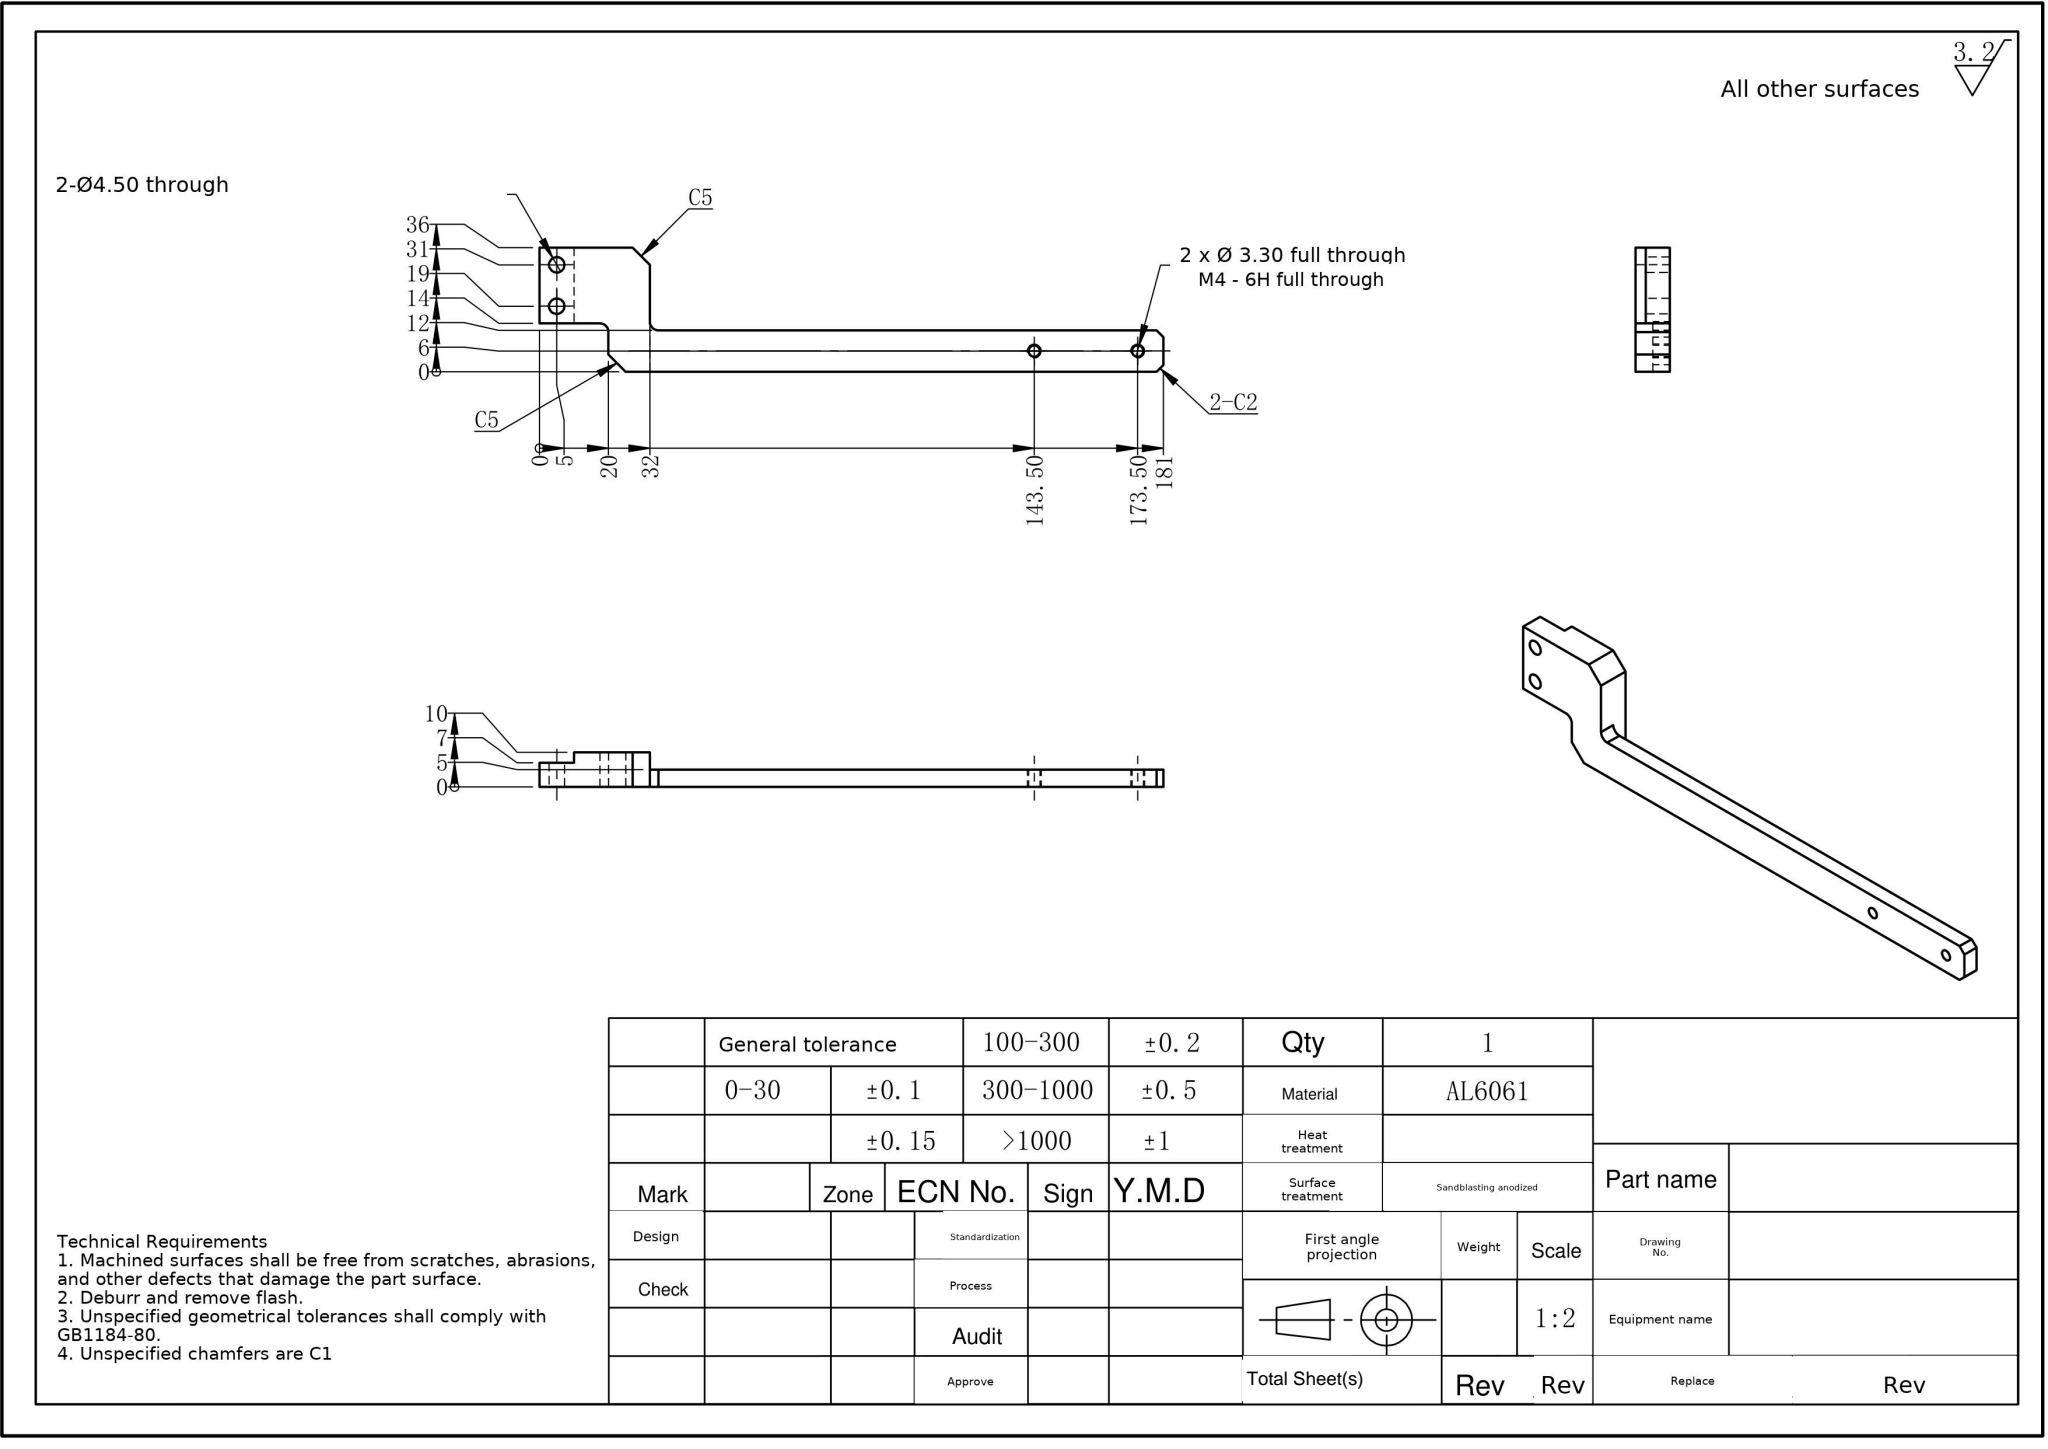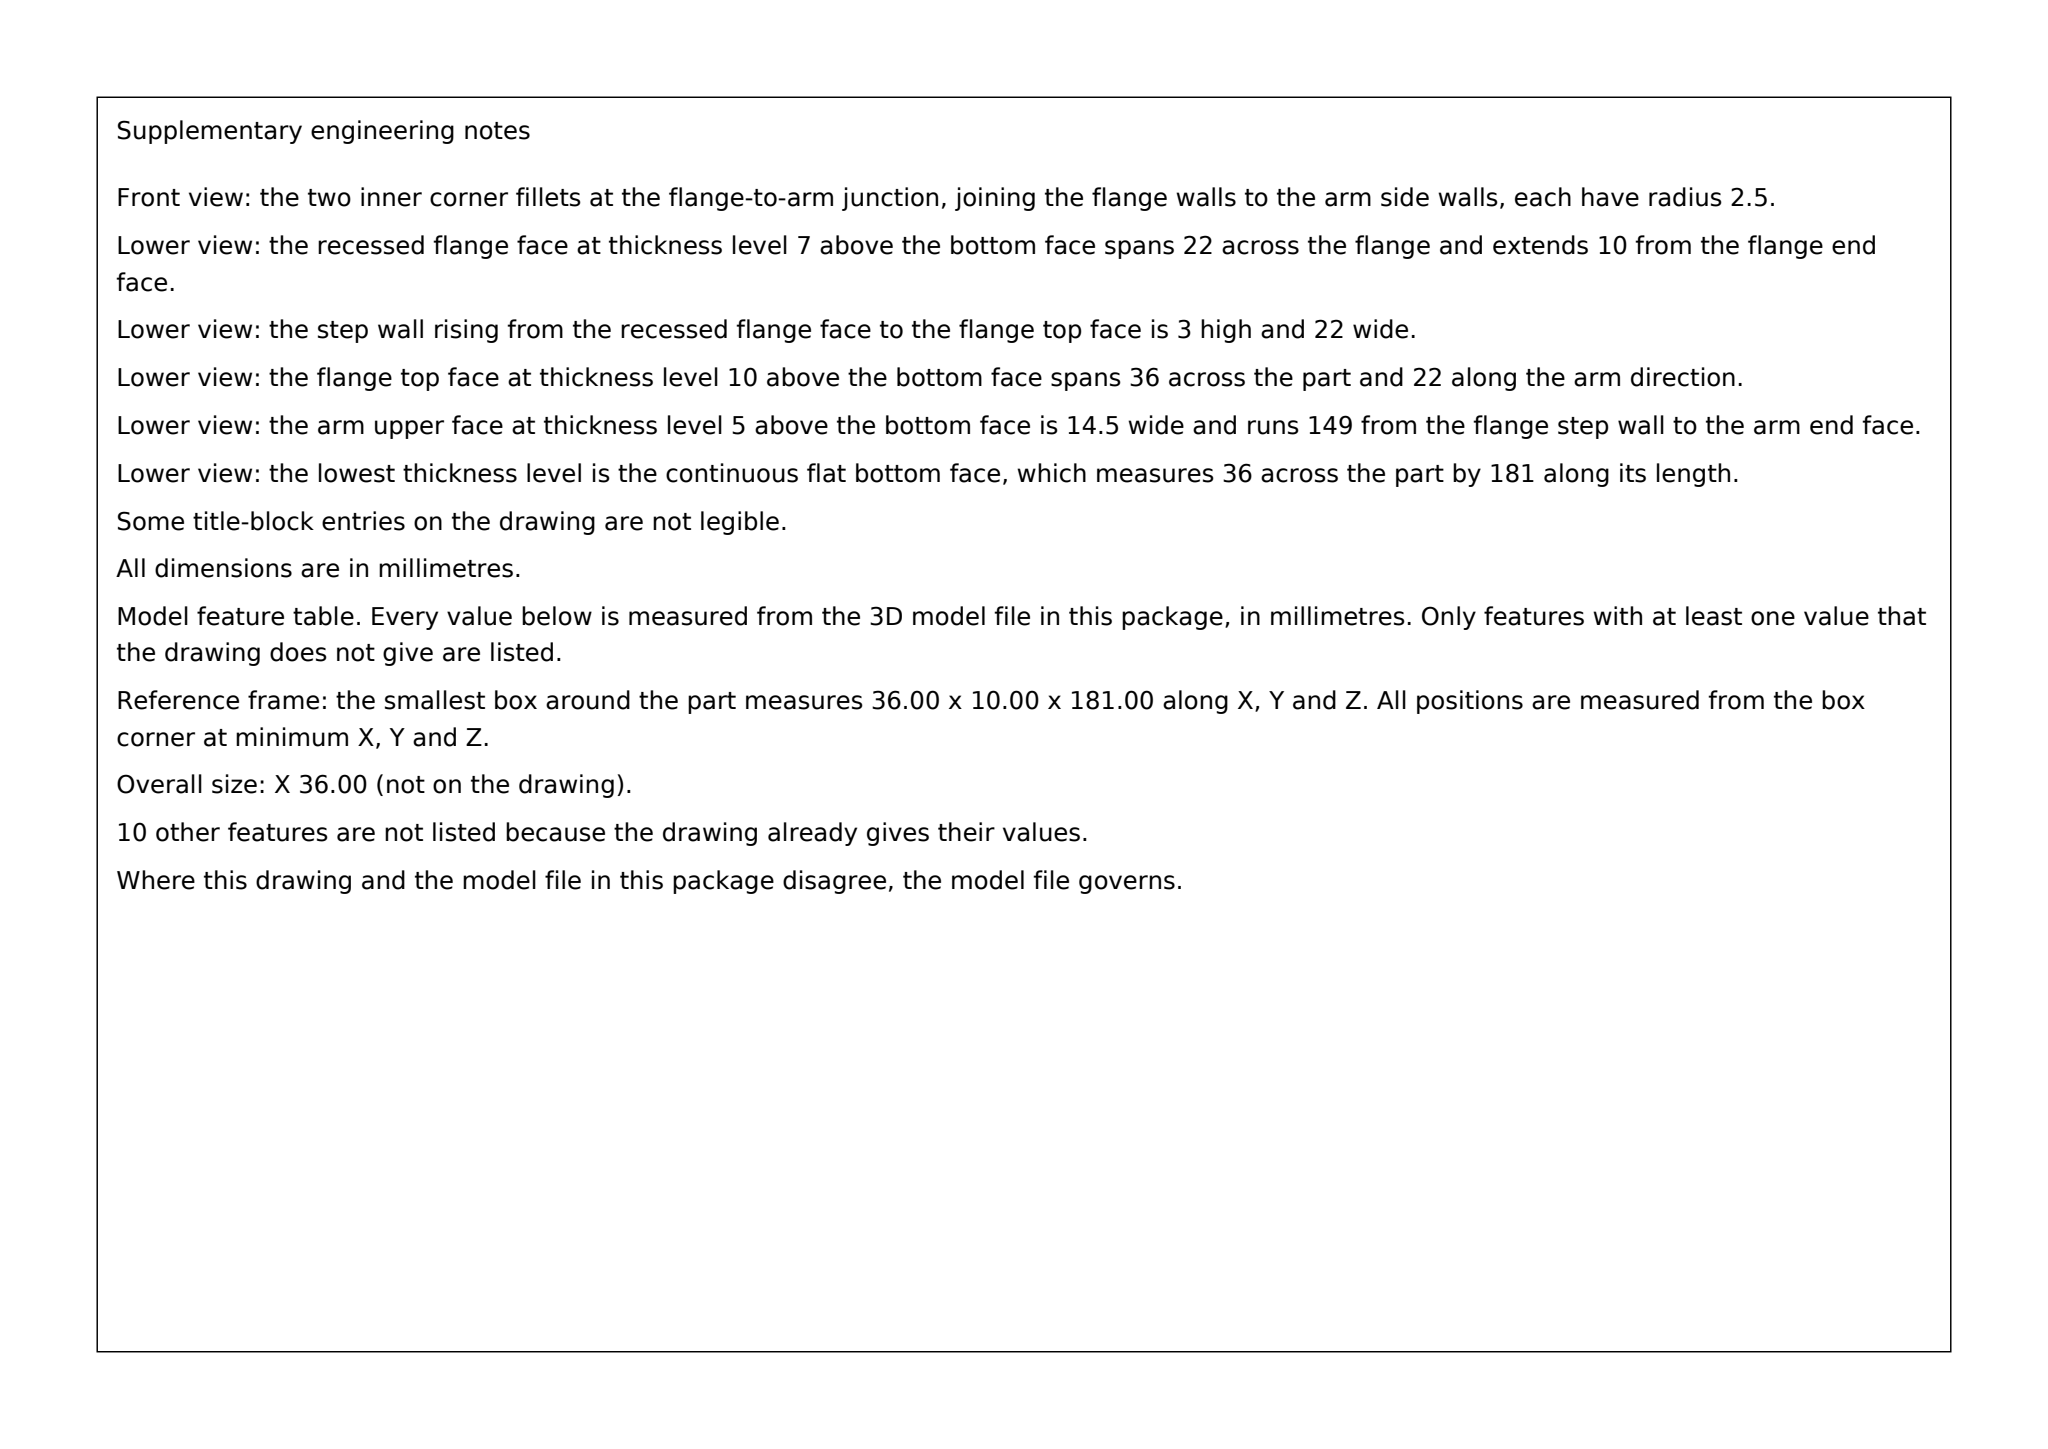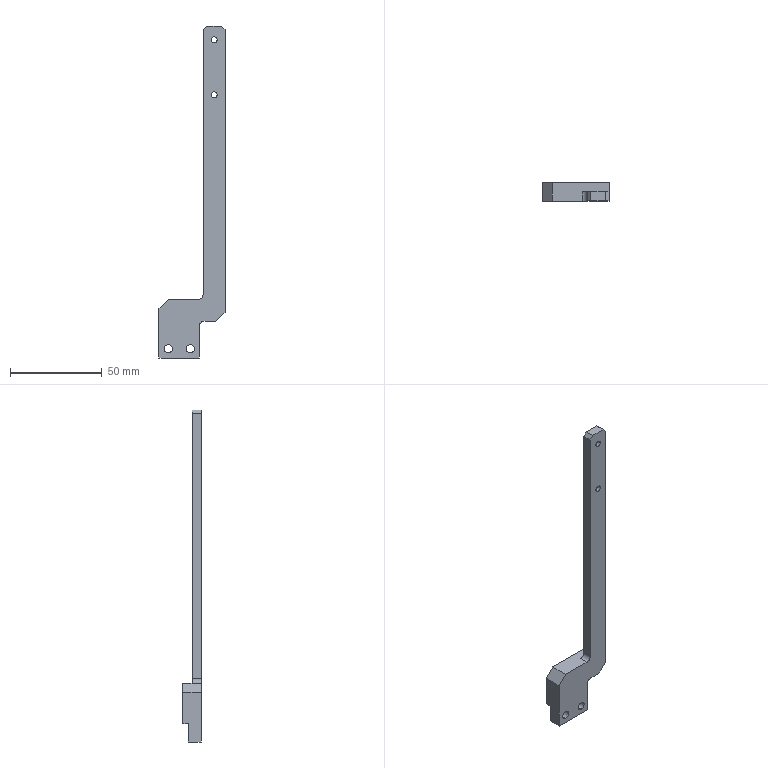Part | SolidWorks | mm | 1 solid | 27 faces | box 36 x 10 x 181 mm | volume 16442 mm3 | plane 17 | cylinder 10 | commonest cylinder face diameters 4.5 x4 3.3 x4 5 x2
Drawing notes:
SIDE VIEW: 7 THK Z0-10, 10 THK Z10-32, 5 THK Z32-181 | from the solid: z planes 0,10,20,32,181; Ø4.5 holes len 7 at z=5 (plate), Ø5 hole len 10 at z=17.5 (boss), Ø3.3 holes len 5 at z=143.5/173.5 and Ø5 len 5 at z=34.5 (arm)
ALL THK STEPS FROM COMMON BTM FACE Y=0; 5 THK ARM STARTS Z=32 | from the solid: y planes 0,5,7,10 only: single datum face y=0 with tops at 5 (arm), 7 (hole plate), 10 (boss); bbox y=10
build123d program:
from build123d import *

# Parameters (mm, degrees)
SKETCH1_W           = 12
SKETCH1_H           = 181
BOSS_EXTRUDE1_DEPTH = 5
SKETCH2_W           = 10
SKETCH2_H           = 3
CUT_EXTRUDE1_DEPTH  = 12
CHAMFER1_SIZE       = 2
M4_TAPPED_HOLE1_D   = 3.3
SKETCH5_W           = 200
SKETCH5_H           = 5
CUT_EXTRUDE2_DEPTH  = 39
BOSS_EXTRUDE3_DEPTH = 24
SKETCH9_W           = 14
SKETCH9_H           = 20
CUT_EXTRUDE4_DEPTH  = 30
CHAMFER2_SIZE       = 5
FILLET1_R           = 2.5
SKETCH10_R          = 2.25
CUT_EXTRUDE5_DEPTH  = 30


with BuildPart() as part:
    # Sketch1 → Boss-Extrude1 (new, symmetric)
    with BuildSketch(Plane(origin=(0, 0, 0), x_dir=(1, 0, 0), z_dir=(0, 1, 0))):
        Rectangle(SKETCH1_W, SKETCH1_H)
    extrude(amount=BOSS_EXTRUDE1_DEPTH, both=True)

    # Sketch2 → Cut-Extrude1 (cut)
    with BuildSketch(Plane(origin=(6, 0, 0), x_dir=(0, 0, -1), z_dir=(1, 0, 0))):
        with Locations((85.5, 3.5)):
            Rectangle(SKETCH2_W, SKETCH2_H)
    extrude(amount=-CUT_EXTRUDE1_DEPTH, mode=Mode.SUBTRACT)

    # Chamfer1
    chamfer1_edges = [part.edges().sort_by_distance(p)[0] for p in [
        (6, 0, 90.5),
        (-6, 0, 90.5),
    ]]
    chamfer(chamfer1_edges, length=CHAMFER1_SIZE)

    # M4 Tapped Hole1 (through all)
    with Locations(Plane(origin=(0, 5, 0), x_dir=(1, 0, 0), z_dir=(0, 1, 0))):
        with Locations((0, -83), (0, -53)):
            Hole(M4_TAPPED_HOLE1_D / 2)

    # Sketch5 → Cut-Extrude2 (cut)
    with BuildSketch(Plane.ZY.offset(6)):
        with Locations((41.5, 2.5)):
            Rectangle(SKETCH5_W, SKETCH5_H)
    extrude(amount=-CUT_EXTRUDE2_DEPTH, mode=Mode.SUBTRACT)

    # Sketch8 → Boss-Extrude3 (add)
    with BuildSketch(Plane.ZY.offset(6)):
        Polygon((-90.5, -5), (-90.5, 2), (-80.5, 2), (-80.5, 5), (-58.5, 5), (-58.5, -5), align=None)
    extrude(amount=BOSS_EXTRUDE3_DEPTH)

    # Sketch9 → Cut-Extrude4 (cut)
    with BuildSketch(Plane(origin=(0, 5, 0), x_dir=(1, 0, 0), z_dir=(0, 1, 0))):
        with Locations((-1, 80.5)):
            Rectangle(SKETCH9_W, SKETCH9_H)
    extrude(amount=-CUT_EXTRUDE4_DEPTH, mode=Mode.SUBTRACT)

    # Chamfer2
    chamfer2_edges = [part.edges().sort_by_distance(p)[0] for p in [
        (6, 0, -70.5),
        (-30, 0, -58.5),
    ]]
    chamfer(chamfer2_edges, length=CHAMFER2_SIZE)

    # Fillet1
    fillet1_edges = [part.edges().sort_by_distance(p)[0] for p in [
        (-8, 0, -70.5),
        (-6, -2.5, -58.5),
    ]]
    fillet(fillet1_edges, radius=FILLET1_R)

    # Sketch10 → Cut-Extrude5 (cut)
    with BuildSketch(Plane(origin=(0, 5, 0), x_dir=(1, 0, 0), z_dir=(0, 1, 0))):
        with Locations(Location((-13, 85.5, 0), (0, 0, 90))):
            Circle(SKETCH10_R)
        with Locations(Location((-25, 85.5, 0), (0, 0, 90))):
            Circle(SKETCH10_R)
    extrude(amount=-CUT_EXTRUDE5_DEPTH, mode=Mode.SUBTRACT)


solid = part.part
STEP:
#1=CARTESIAN_POINT('',(-25.,-5.,-83.25));
#2=VERTEX_POINT('',#1);
#3=CARTESIAN_POINT('',(-25.,-5.,-87.75));
#4=VERTEX_POINT('',#3);
#5=CARTESIAN_POINT('',(-25.,-5.,-85.5));
#6=DIRECTION('',(0.,-1.,0.));
#7=DIRECTION('',(0.,0.,-1.));
#8=AXIS2_PLACEMENT_3D('',#5,#6,#7);
#9=CIRCLE('',#8,2.25);
#10=EDGE_CURVE('',#2,#4,#9,.T.);
#11=ORIENTED_EDGE('',*,*,#10,.T.);
#12=CARTESIAN_POINT('',(-25.,2.,-87.75));
#13=VERTEX_POINT('',#12);
#14=CARTESIAN_POINT('',(-25.,-25.,-87.75));
#15=DIRECTION('',(0.,1.,0.));
#16=VECTOR('',#15,1000.);
#17=LINE('',#14,#16);
#18=EDGE_CURVE('',#4,#13,#17,.T.);
#19=ORIENTED_EDGE('',*,*,#18,.T.);
#20=CARTESIAN_POINT('',(-25.,2.,-83.25));
#21=VERTEX_POINT('',#20);
#22=CARTESIAN_POINT('',(-25.,2.,-85.5));
#23=DIRECTION('',(0.,-1.,-0.));
#24=DIRECTION('',(0.,0.,-1.));
#25=AXIS2_PLACEMENT_3D('',#22,#23,#24);
#26=CIRCLE('',#25,2.25);
#27=EDGE_CURVE('',#21,#13,#26,.T.);
#28=ORIENTED_EDGE('',*,*,#27,.F.);
#29=CARTESIAN_POINT('',(-25.,-25.,-83.25));
#30=DIRECTION('',(0.,1.,0.));
#31=VECTOR('',#30,1000.);
#32=LINE('',#29,#31);
#33=EDGE_CURVE('',#2,#21,#32,.T.);
#34=ORIENTED_EDGE('',*,*,#33,.F.);
#35=EDGE_LOOP('',(#11,#19,#28,#34));
#36=FACE_OUTER_BOUND('',#35,.T.);
#37=CARTESIAN_POINT('',(-25.,-25.,-85.5));
#38=DIRECTION('',(0.,1.,0.));
#39=DIRECTION('',(0.,0.,1.));
#40=AXIS2_PLACEMENT_3D('',#37,#38,#39);
#41=CYLINDRICAL_SURFACE('',#40,2.25);
#42=ADVANCED_FACE('',(#36),#41,.F.);
#43=CARTESIAN_POINT('',(-13.,-5.,-83.25));
#44=VERTEX_POINT('',#43);
#45=CARTESIAN_POINT('',(-13.,-5.,-87.75));
#46=VERTEX_POINT('',#45);
#47=CARTESIAN_POINT('',(-13.,-5.,-85.5));
#48=DIRECTION('',(0.,-1.,0.));
#49=DIRECTION('',(0.,0.,-1.));
#50=AXIS2_PLACEMENT_3D('',#47,#48,#49);
#51=CIRCLE('',#50,2.25);
#52=EDGE_CURVE('',#44,#46,#51,.T.);
#53=ORIENTED_EDGE('',*,*,#52,.T.);
#54=CARTESIAN_POINT('',(-13.,2.,-87.75));
#55=VERTEX_POINT('',#54);
#56=CARTESIAN_POINT('',(-13.,-25.,-87.75));
#57=DIRECTION('',(0.,1.,0.));
#58=VECTOR('',#57,1000.);
#59=LINE('',#56,#58);
#60=EDGE_CURVE('',#46,#55,#59,.T.);
#61=ORIENTED_EDGE('',*,*,#60,.T.);
#62=CARTESIAN_POINT('',(-13.,2.,-83.25));
#63=VERTEX_POINT('',#62);
#64=CARTESIAN_POINT('',(-13.,2.,-85.5));
#65=DIRECTION('',(0.,-1.,-0.));
#66=DIRECTION('',(0.,0.,-1.));
#67=AXIS2_PLACEMENT_3D('',#64,#65,#66);
#68=CIRCLE('',#67,2.25);
#69=EDGE_CURVE('',#63,#55,#68,.T.);
#70=ORIENTED_EDGE('',*,*,#69,.F.);
#71=CARTESIAN_POINT('',(-13.,-25.,-83.25));
#72=DIRECTION('',(0.,1.,0.));
#73=VECTOR('',#72,1000.);
#74=LINE('',#71,#73);
#75=EDGE_CURVE('',#44,#63,#74,.T.);
#76=ORIENTED_EDGE('',*,*,#75,.F.);
#77=EDGE_LOOP('',(#53,#61,#70,#76));
#78=FACE_OUTER_BOUND('',#77,.T.);
#79=CARTESIAN_POINT('',(-13.,-25.,-85.5));
#80=DIRECTION('',(0.,1.,0.));
#81=DIRECTION('',(0.,0.,1.));
#82=AXIS2_PLACEMENT_3D('',#79,#80,#81);
#83=CYLINDRICAL_SURFACE('',#82,2.25);
#84=ADVANCED_FACE('',(#78),#83,.F.);
#85=CARTESIAN_POINT('',(0.,-5.,81.35));
#86=VERTEX_POINT('',#85);
#87=CARTESIAN_POINT('',(0.,-5.,84.65));
#88=VERTEX_POINT('',#87);
#89=CARTESIAN_POINT('',(0.,-5.,83.));
#90=DIRECTION('',(0.,1.,0.));
#91=DIRECTION('',(0.,0.,1.));
#92=AXIS2_PLACEMENT_3D('',#89,#90,#91);
#93=CIRCLE('',#92,1.65);
#94=EDGE_CURVE('',#86,#88,#93,.T.);
#95=ORIENTED_EDGE('',*,*,#94,.F.);
#96=CARTESIAN_POINT('',(0.,-0.,81.35));
#97=VERTEX_POINT('',#96);
#98=CARTESIAN_POINT('',(0.,5.,81.35));
#99=DIRECTION('',(0.,1.,0.));
#100=VECTOR('',#99,1000.);
#101=LINE('',#98,#100);
#102=EDGE_CURVE('',#86,#97,#101,.T.);
#103=ORIENTED_EDGE('',*,*,#102,.T.);
#104=CARTESIAN_POINT('',(0.,-0.,84.65));
#105=VERTEX_POINT('',#104);
#106=CARTESIAN_POINT('',(0.,-0.,83.));
#107=DIRECTION('',(0.,1.,-0.));
#108=DIRECTION('',(0.,-0.,-1.));
#109=AXIS2_PLACEMENT_3D('',#106,#107,#108);
#110=CIRCLE('',#109,1.65);
#111=EDGE_CURVE('',#97,#105,#110,.T.);
#112=ORIENTED_EDGE('',*,*,#111,.T.);
#113=CARTESIAN_POINT('',(0.,5.,84.65));
#114=DIRECTION('',(0.,1.,0.));
#115=VECTOR('',#114,1000.);
#116=LINE('',#113,#115);
#117=EDGE_CURVE('',#88,#105,#116,.T.);
#118=ORIENTED_EDGE('',*,*,#117,.F.);
#119=EDGE_LOOP('',(#95,#103,#112,#118));
#120=FACE_OUTER_BOUND('',#119,.T.);
#121=CARTESIAN_POINT('',(0.,5.,83.));
#122=DIRECTION('',(0.,1.,0.));
#123=DIRECTION('',(0.,0.,1.));
#124=AXIS2_PLACEMENT_3D('',#121,#122,#123);
#125=CYLINDRICAL_SURFACE('',#124,1.65);
#126=ADVANCED_FACE('',(#120),#125,.F.);
#127=CARTESIAN_POINT('',(0.,-5.,51.35));
#128=VERTEX_POINT('',#127);
#129=CARTESIAN_POINT('',(0.,-5.,54.65));
#130=VERTEX_POINT('',#129);
#131=CARTESIAN_POINT('',(0.,-5.,53.));
#132=DIRECTION('',(0.,1.,0.));
#133=DIRECTION('',(0.,0.,1.));
#134=AXIS2_PLACEMENT_3D('',#131,#132,#133);
#135=CIRCLE('',#134,1.65);
#136=EDGE_CURVE('',#128,#130,#135,.T.);
#137=ORIENTED_EDGE('',*,*,#136,.F.);
#138=CARTESIAN_POINT('',(0.,-0.,51.35));
#139=VERTEX_POINT('',#138);
#140=CARTESIAN_POINT('',(0.,5.,51.35));
#141=DIRECTION('',(0.,1.,0.));
#142=VECTOR('',#141,1000.);
#143=LINE('',#140,#142);
#144=EDGE_CURVE('',#128,#139,#143,.T.);
#145=ORIENTED_EDGE('',*,*,#144,.T.);
#146=CARTESIAN_POINT('',(0.,-0.,54.65));
#147=VERTEX_POINT('',#146);
#148=CARTESIAN_POINT('',(0.,-0.,53.));
#149=DIRECTION('',(0.,1.,-0.));
#150=DIRECTION('',(0.,-0.,-1.));
#151=AXIS2_PLACEMENT_3D('',#148,#149,#150);
#152=CIRCLE('',#151,1.65);
#153=EDGE_CURVE('',#139,#147,#152,.T.);
#154=ORIENTED_EDGE('',*,*,#153,.T.);
#155=CARTESIAN_POINT('',(0.,5.,54.65));
#156=DIRECTION('',(0.,1.,0.));
#157=VECTOR('',#156,1000.);
#158=LINE('',#155,#157);
#159=EDGE_CURVE('',#130,#147,#158,.T.);
#160=ORIENTED_EDGE('',*,*,#159,.F.);
#161=EDGE_LOOP('',(#137,#145,#154,#160));
#162=FACE_OUTER_BOUND('',#161,.T.);
#163=CARTESIAN_POINT('',(0.,5.,53.));
#164=DIRECTION('',(0.,1.,0.));
#165=DIRECTION('',(0.,0.,1.));
#166=AXIS2_PLACEMENT_3D('',#163,#164,#165);
#167=CYLINDRICAL_SURFACE('',#166,1.65);
#168=ADVANCED_FACE('',(#162),#167,.F.);
#169=CARTESIAN_POINT('',(-6.,-0.,-56.));
#170=VERTEX_POINT('',#169);
#171=CARTESIAN_POINT('',(-6.,-0.,88.5));
#172=VERTEX_POINT('',#171);
#173=CARTESIAN_POINT('',(-6.,0.,141.5));
#174=DIRECTION('',(0.,0.,1.));
#175=VECTOR('',#174,1000.);
#176=LINE('',#173,#175);
#177=EDGE_CURVE('',#170,#172,#176,.T.);
#178=ORIENTED_EDGE('',*,*,#177,.F.);
#179=CARTESIAN_POINT('',(-6.,-5.,-56.));
#180=VERTEX_POINT('',#179);
#181=CARTESIAN_POINT('',(-6.,-5.,-56.));
#182=DIRECTION('',(0.,-1.,0.));
#183=VECTOR('',#182,1000.);
#184=LINE('',#181,#183);
#185=EDGE_CURVE('',#170,#180,#184,.T.);
#186=ORIENTED_EDGE('',*,*,#185,.T.);
#187=CARTESIAN_POINT('',(-6.,-5.,88.5));
#188=VERTEX_POINT('',#187);
#189=CARTESIAN_POINT('',(-6.,-5.,90.5));
#190=DIRECTION('',(0.,0.,1.));
#191=VECTOR('',#190,1000.);
#192=LINE('',#189,#191);
#193=EDGE_CURVE('',#180,#188,#192,.T.);
#194=ORIENTED_EDGE('',*,*,#193,.T.);
#195=CARTESIAN_POINT('',(-6.,5.,88.5));
#196=DIRECTION('',(0.,1.,0.));
#197=VECTOR('',#196,1000.);
#198=LINE('',#195,#197);
#199=EDGE_CURVE('',#188,#172,#198,.T.);
#200=ORIENTED_EDGE('',*,*,#199,.T.);
#201=EDGE_LOOP('',(#178,#186,#194,#200));
#202=FACE_OUTER_BOUND('',#201,.T.);
#203=CARTESIAN_POINT('',(-6.,5.,90.5));
#204=DIRECTION('',(1.,0.,0.));
#205=DIRECTION('',(0.,0.,-1.));
#206=AXIS2_PLACEMENT_3D('',#203,#204,#205);
#207=PLANE('',#206);
#208=ADVANCED_FACE('',(#202),#207,.F.);
#209=CARTESIAN_POINT('',(-30.,5.,-63.5));
#210=VERTEX_POINT('',#209);
#211=CARTESIAN_POINT('',(-30.,5.,-80.5));
#212=VERTEX_POINT('',#211);
#213=CARTESIAN_POINT('',(-30.,5.,-80.5));
#214=DIRECTION('',(0.,0.,-1.));
#215=VECTOR('',#214,1000.);
#216=LINE('',#213,#215);
#217=EDGE_CURVE('',#210,#212,#216,.T.);
#218=ORIENTED_EDGE('',*,*,#217,.F.);
#219=CARTESIAN_POINT('',(-25.,5.,-58.5));
#220=VERTEX_POINT('',#219);
#221=CARTESIAN_POINT('',(-30.,5.,-63.5));
#222=DIRECTION('',(0.7071,0.,0.7071));
#223=VECTOR('',#222,1000.);
#224=LINE('',#221,#223);
#225=EDGE_CURVE('',#210,#220,#224,.T.);
#226=ORIENTED_EDGE('',*,*,#225,.T.);
#227=CARTESIAN_POINT('',(6.,5.,-58.5));
#228=VERTEX_POINT('',#227);
#229=CARTESIAN_POINT('',(33.,5.,-58.5));
#230=DIRECTION('',(-1.,0.,0.));
#231=VECTOR('',#230,1000.);
#232=LINE('',#229,#231);
#233=EDGE_CURVE('',#228,#220,#232,.T.);
#234=ORIENTED_EDGE('',*,*,#233,.F.);
#235=CARTESIAN_POINT('',(6.,5.,-65.5));
#236=VERTEX_POINT('',#235);
#237=CARTESIAN_POINT('',(6.,5.,90.5));
#238=DIRECTION('',(0.,0.,-1.));
#239=VECTOR('',#238,1000.);
#240=LINE('',#237,#239);
#241=EDGE_CURVE('',#228,#236,#240,.T.);
#242=ORIENTED_EDGE('',*,*,#241,.T.);
#243=CARTESIAN_POINT('',(1.,5.,-70.5));
#244=VERTEX_POINT('',#243);
#245=CARTESIAN_POINT('',(6.,5.,-65.5));
#246=DIRECTION('',(-0.7071,0.,-0.7071));
#247=VECTOR('',#246,1000.);
#248=LINE('',#245,#247);
#249=EDGE_CURVE('',#236,#244,#248,.T.);
#250=ORIENTED_EDGE('',*,*,#249,.T.);
#251=CARTESIAN_POINT('',(-5.5,5.,-70.5));
#252=VERTEX_POINT('',#251);
#253=CARTESIAN_POINT('',(6.,5.,-70.5));
#254=DIRECTION('',(1.,0.,0.));
#255=VECTOR('',#254,1000.);
#256=LINE('',#253,#255);
#257=EDGE_CURVE('',#252,#244,#256,.T.);
#258=ORIENTED_EDGE('',*,*,#257,.F.);
#259=CARTESIAN_POINT('',(-8.,5.,-73.));
#260=VERTEX_POINT('',#259);
#261=CARTESIAN_POINT('',(-5.5,5.,-73.));
#262=DIRECTION('',(0.,-1.,0.));
#263=DIRECTION('',(0.,0.,-1.));
#264=AXIS2_PLACEMENT_3D('',#261,#262,#263);
#265=CIRCLE('',#264,2.5);
#266=EDGE_CURVE('',#252,#260,#265,.T.);
#267=ORIENTED_EDGE('',*,*,#266,.T.);
#268=CARTESIAN_POINT('',(-8.,5.,-80.5));
#269=VERTEX_POINT('',#268);
#270=CARTESIAN_POINT('',(-8.,5.,-70.5));
#271=DIRECTION('',(0.,0.,1.));
#272=VECTOR('',#271,1000.);
#273=LINE('',#270,#272);
#274=EDGE_CURVE('',#269,#260,#273,.T.);
#275=ORIENTED_EDGE('',*,*,#274,.F.);
#276=CARTESIAN_POINT('',(-16.44,5.,-80.5));
#277=DIRECTION('',(1.,0.,0.));
#278=VECTOR('',#277,1000.);
#279=LINE('',#276,#278);
#280=EDGE_CURVE('',#212,#269,#279,.T.);
#281=ORIENTED_EDGE('',*,*,#280,.F.);
#282=EDGE_LOOP('',(#218,#226,#234,#242,#250,#258,#267,#275,#281));
#283=FACE_OUTER_BOUND('',#282,.T.);
#284=CARTESIAN_POINT('',(0.,5.,0.));
#285=DIRECTION('',(0.,-1.,0.));
#286=DIRECTION('',(0.,0.,-1.));
#287=AXIS2_PLACEMENT_3D('',#284,#285,#286);
#288=PLANE('',#287);
#289=ADVANCED_FACE('',(#283),#288,.F.);
#290=CARTESIAN_POINT('',(6.,-5.,88.5));
#291=VERTEX_POINT('',#290);
#292=CARTESIAN_POINT('',(6.,-5.,-65.5));
#293=VERTEX_POINT('',#292);
#294=CARTESIAN_POINT('',(6.,-5.,90.5));
#295=DIRECTION('',(0.,0.,-1.));
#296=VECTOR('',#295,1000.);
#297=LINE('',#294,#296);
#298=EDGE_CURVE('',#291,#293,#297,.T.);
#299=ORIENTED_EDGE('',*,*,#298,.T.);
#300=CARTESIAN_POINT('',(6.,5.,-65.5));
#301=DIRECTION('',(0.,1.,0.));
#302=VECTOR('',#301,1000.);
#303=LINE('',#300,#302);
#304=EDGE_CURVE('',#293,#236,#303,.T.);
#305=ORIENTED_EDGE('',*,*,#304,.T.);
#306=ORIENTED_EDGE('',*,*,#241,.F.);
#307=CARTESIAN_POINT('',(6.,-0.,-58.5));
#308=VERTEX_POINT('',#307);
#309=CARTESIAN_POINT('',(6.,5.,-58.5));
#310=DIRECTION('',(0.,-1.,0.));
#311=VECTOR('',#310,1000.);
#312=LINE('',#309,#311);
#313=EDGE_CURVE('',#228,#308,#312,.T.);
#314=ORIENTED_EDGE('',*,*,#313,.T.);
#315=CARTESIAN_POINT('',(6.,-0.,88.5));
#316=VERTEX_POINT('',#315);
#317=CARTESIAN_POINT('',(6.,-0.,90.5));
#318=DIRECTION('',(0.,0.,1.));
#319=VECTOR('',#318,1000.);
#320=LINE('',#317,#319);
#321=EDGE_CURVE('',#308,#316,#320,.T.);
#322=ORIENTED_EDGE('',*,*,#321,.T.);
#323=CARTESIAN_POINT('',(6.,5.,88.5));
#324=DIRECTION('',(0.,-1.,0.));
#325=VECTOR('',#324,1000.);
#326=LINE('',#323,#325);
#327=EDGE_CURVE('',#316,#291,#326,.T.);
#328=ORIENTED_EDGE('',*,*,#327,.T.);
#329=EDGE_LOOP('',(#299,#305,#306,#314,#322,#328));
#330=FACE_OUTER_BOUND('',#329,.T.);
#331=CARTESIAN_POINT('',(6.,5.,90.5));
#332=DIRECTION('',(-1.,0.,0.));
#333=DIRECTION('',(0.,0.,1.));
#334=AXIS2_PLACEMENT_3D('',#331,#332,#333);
#335=PLANE('',#334);
#336=ADVANCED_FACE('',(#330),#335,.F.);
#337=CARTESIAN_POINT('',(-30.,2.,-90.5));
#338=VERTEX_POINT('',#337);
#339=CARTESIAN_POINT('',(-8.,2.,-90.5));
#340=VERTEX_POINT('',#339);
#341=CARTESIAN_POINT('',(-16.44,2.,-90.5));
#342=DIRECTION('',(1.,0.,0.));
#343=VECTOR('',#342,1000.);
#344=LINE('',#341,#343);
#345=EDGE_CURVE('',#338,#340,#344,.T.);
#346=ORIENTED_EDGE('',*,*,#345,.T.);
#347=CARTESIAN_POINT('',(-8.,-5.,-90.5));
#348=VERTEX_POINT('',#347);
#349=CARTESIAN_POINT('',(-8.,-25.,-90.5));
#350=DIRECTION('',(0.,1.,0.));
#351=VECTOR('',#350,1000.);
#352=LINE('',#349,#351);
#353=EDGE_CURVE('',#348,#340,#352,.T.);
#354=ORIENTED_EDGE('',*,*,#353,.F.);
#355=CARTESIAN_POINT('',(-30.,-5.,-90.5));
#356=VERTEX_POINT('',#355);
#357=CARTESIAN_POINT('',(-6.,-5.,-90.5));
#358=DIRECTION('',(-1.,0.,0.));
#359=VECTOR('',#358,1000.);
#360=LINE('',#357,#359);
#361=EDGE_CURVE('',#348,#356,#360,.T.);
#362=ORIENTED_EDGE('',*,*,#361,.T.);
#363=CARTESIAN_POINT('',(-30.,-5.,-90.5));
#364=DIRECTION('',(0.,-1.,0.));
#365=VECTOR('',#364,1000.);
#366=LINE('',#363,#365);
#367=EDGE_CURVE('',#338,#356,#366,.T.);
#368=ORIENTED_EDGE('',*,*,#367,.F.);
#369=EDGE_LOOP('',(#346,#354,#362,#368));
#370=FACE_OUTER_BOUND('',#369,.T.);
#371=CARTESIAN_POINT('',(-6.,5.,-90.5));
#372=DIRECTION('',(0.,0.,1.));
#373=DIRECTION('',(1.,0.,0.));
#374=AXIS2_PLACEMENT_3D('',#371,#372,#373);
#375=PLANE('',#374);
#376=ADVANCED_FACE('',(#370),#375,.F.);
#377=CARTESIAN_POINT('',(4.,-5.,90.5));
#378=VERTEX_POINT('',#377);
#379=CARTESIAN_POINT('',(4.,-0.,90.5));
#380=VERTEX_POINT('',#379);
#381=CARTESIAN_POINT('',(4.,5.,90.5));
#382=DIRECTION('',(0.,1.,0.));
#383=VECTOR('',#382,1000.);
#384=LINE('',#381,#383);
#385=EDGE_CURVE('',#378,#380,#384,.T.);
#386=ORIENTED_EDGE('',*,*,#385,.T.);
#387=CARTESIAN_POINT('',(-4.,-0.,90.5));
#388=VERTEX_POINT('',#387);
#389=CARTESIAN_POINT('',(-6.,-0.,90.5));
#390=DIRECTION('',(-1.,0.,0.));
#391=VECTOR('',#390,1000.);
#392=LINE('',#389,#391);
#393=EDGE_CURVE('',#380,#388,#392,.T.);
#394=ORIENTED_EDGE('',*,*,#393,.T.);
#395=CARTESIAN_POINT('',(-4.,-5.,90.5));
#396=VERTEX_POINT('',#395);
#397=CARTESIAN_POINT('',(-4.,5.,90.5));
#398=DIRECTION('',(0.,-1.,0.));
#399=VECTOR('',#398,1000.);
#400=LINE('',#397,#399);
#401=EDGE_CURVE('',#388,#396,#400,.T.);
#402=ORIENTED_EDGE('',*,*,#401,.T.);
#403=CARTESIAN_POINT('',(-6.,-5.,90.5));
#404=DIRECTION('',(1.,0.,0.));
#405=VECTOR('',#404,1000.);
#406=LINE('',#403,#405);
#407=EDGE_CURVE('',#396,#378,#406,.T.);
#408=ORIENTED_EDGE('',*,*,#407,.T.);
#409=EDGE_LOOP('',(#386,#394,#402,#408));
#410=FACE_OUTER_BOUND('',#409,.T.);
#411=CARTESIAN_POINT('',(-6.,5.,90.5));
#412=DIRECTION('',(0.,0.,-1.));
#413=DIRECTION('',(-1.,0.,0.));
#414=AXIS2_PLACEMENT_3D('',#411,#412,#413);
#415=PLANE('',#414);
#416=ADVANCED_FACE('',(#410),#415,.F.);
#417=ORIENTED_EDGE('',*,*,#10,.F.);
#418=CARTESIAN_POINT('',(-25.,-5.,-85.5));
#419=DIRECTION('',(0.,-1.,0.));
#420=DIRECTION('',(0.,0.,-1.));
#421=AXIS2_PLACEMENT_3D('',#418,#419,#420);
#422=CIRCLE('',#421,2.25);
#423=EDGE_CURVE('',#4,#2,#422,.T.);
#424=ORIENTED_EDGE('',*,*,#423,.F.);
#425=EDGE_LOOP('',(#417,#424));
#426=FACE_BOUND('',#425,.T.);
#427=ORIENTED_EDGE('',*,*,#52,.F.);
#428=CARTESIAN_POINT('',(-13.,-5.,-85.5));
#429=DIRECTION('',(0.,-1.,0.));
#430=DIRECTION('',(0.,0.,-1.));
#431=AXIS2_PLACEMENT_3D('',#428,#429,#430);
#432=CIRCLE('',#431,2.25);
#433=EDGE_CURVE('',#46,#44,#432,.T.);
#434=ORIENTED_EDGE('',*,*,#433,.F.);
#435=EDGE_LOOP('',(#427,#434));
#436=FACE_BOUND('',#435,.T.);
#437=CARTESIAN_POINT('',(-25.,-5.,-58.5));
#438=VERTEX_POINT('',#437);
#439=CARTESIAN_POINT('',(-8.5,-5.,-58.5));
#440=VERTEX_POINT('',#439);
#441=CARTESIAN_POINT('',(-30.,-5.,-58.5));
#442=DIRECTION('',(1.,0.,0.));
#443=VECTOR('',#442,1000.);
#444=LINE('',#441,#443);
#445=EDGE_CURVE('',#438,#440,#444,.T.);
#446=ORIENTED_EDGE('',*,*,#445,.F.);
#447=CARTESIAN_POINT('',(-30.,-5.,-63.5));
#448=VERTEX_POINT('',#447);
#449=CARTESIAN_POINT('',(16.75,-5.,-16.75));
#450=DIRECTION('',(-0.7071,0.,-0.7071));
#451=VECTOR('',#450,1000.);
#452=LINE('',#449,#451);
#453=EDGE_CURVE('',#438,#448,#452,.T.);
#454=ORIENTED_EDGE('',*,*,#453,.T.);
#455=CARTESIAN_POINT('',(-30.,-5.,-58.5));
#456=DIRECTION('',(0.,-0.,1.));
#457=VECTOR('',#456,1000.);
#458=LINE('',#455,#457);
#459=EDGE_CURVE('',#356,#448,#458,.T.);
#460=ORIENTED_EDGE('',*,*,#459,.F.);
#461=ORIENTED_EDGE('',*,*,#361,.F.);
#462=CARTESIAN_POINT('',(-8.,-5.,-73.));
#463=VERTEX_POINT('',#462);
#464=CARTESIAN_POINT('',(-8.,-5.,0.));
#465=DIRECTION('',(0.,0.,-1.));
#466=VECTOR('',#465,1000.);
#467=LINE('',#464,#466);
#468=EDGE_CURVE('',#463,#348,#467,.T.);
#469=ORIENTED_EDGE('',*,*,#468,.F.);
#470=CARTESIAN_POINT('',(-5.5,-5.,-70.5));
#471=VERTEX_POINT('',#470);
#472=CARTESIAN_POINT('',(-5.5,-5.,-73.));
#473=DIRECTION('',(0.,1.,0.));
#474=DIRECTION('',(0.,0.,-1.));
#475=AXIS2_PLACEMENT_3D('',#472,#473,#474);
#476=CIRCLE('',#475,2.5);
#477=EDGE_CURVE('',#463,#471,#476,.T.);
#478=ORIENTED_EDGE('',*,*,#477,.T.);
#479=CARTESIAN_POINT('',(1.,-5.,-70.5));
#480=VERTEX_POINT('',#479);
#481=CARTESIAN_POINT('',(0.,-5.,-70.5));
#482=DIRECTION('',(-1.,0.,0.));
#483=VECTOR('',#482,1000.);
#484=LINE('',#481,#483);
#485=EDGE_CURVE('',#480,#471,#484,.T.);
#486=ORIENTED_EDGE('',*,*,#485,.F.);
#487=CARTESIAN_POINT('',(35.75,-5.,-35.75));
#488=DIRECTION('',(0.7071,0.,0.7071));
#489=VECTOR('',#488,1000.);
#490=LINE('',#487,#489);
#491=EDGE_CURVE('',#480,#293,#490,.T.);
#492=ORIENTED_EDGE('',*,*,#491,.T.);
#493=ORIENTED_EDGE('',*,*,#298,.F.);
#494=CARTESIAN_POINT('',(47.25,-5.,47.25));
#495=DIRECTION('',(-0.7071,0.,0.7071));
#496=VECTOR('',#495,1000.);
#497=LINE('',#494,#496);
#498=EDGE_CURVE('',#291,#378,#497,.T.);
#499=ORIENTED_EDGE('',*,*,#498,.T.);
#500=ORIENTED_EDGE('',*,*,#407,.F.);
#501=CARTESIAN_POINT('',(-47.25,-5.,47.25));
#502=DIRECTION('',(-0.7071,0.,-0.7071));
#503=VECTOR('',#502,1000.);
#504=LINE('',#501,#503);
#505=EDGE_CURVE('',#396,#188,#504,.T.);
#506=ORIENTED_EDGE('',*,*,#505,.T.);
#507=ORIENTED_EDGE('',*,*,#193,.F.);
#508=CARTESIAN_POINT('',(-8.5,-5.,-56.));
#509=DIRECTION('',(0.,1.,0.));
#510=DIRECTION('',(0.,0.,-1.));
#511=AXIS2_PLACEMENT_3D('',#508,#509,#510);
#512=CIRCLE('',#511,2.5);
#513=EDGE_CURVE('',#180,#440,#512,.T.);
#514=ORIENTED_EDGE('',*,*,#513,.T.);
#515=EDGE_LOOP('',(#446,#454,#460,#461,#469,#478,#486,#492,#493,#499,#500,#506,#507,#514));
#516=FACE_OUTER_BOUND('',#515,.T.);
#517=CARTESIAN_POINT('',(0.,-5.,83.));
#518=DIRECTION('',(0.,1.,0.));
#519=DIRECTION('',(0.,0.,1.));
#520=AXIS2_PLACEMENT_3D('',#517,#518,#519);
#521=CIRCLE('',#520,1.65);
#522=EDGE_CURVE('',#88,#86,#521,.T.);
#523=ORIENTED_EDGE('',*,*,#522,.T.);
#524=ORIENTED_EDGE('',*,*,#94,.T.);
#525=EDGE_LOOP('',(#523,#524));
#526=FACE_BOUND('',#525,.T.);
#527=CARTESIAN_POINT('',(0.,-5.,53.));
#528=DIRECTION('',(0.,1.,0.));
#529=DIRECTION('',(0.,0.,1.));
#530=AXIS2_PLACEMENT_3D('',#527,#528,#529);
#531=CIRCLE('',#530,1.65);
#532=EDGE_CURVE('',#130,#128,#531,.T.);
#533=ORIENTED_EDGE('',*,*,#532,.T.);
#534=ORIENTED_EDGE('',*,*,#136,.T.);
#535=EDGE_LOOP('',(#533,#534));
#536=FACE_BOUND('',#535,.T.);
#537=CARTESIAN_POINT('',(0.,-5.,0.));
#538=DIRECTION('',(0.,-1.,0.));
#539=DIRECTION('',(0.,0.,-1.));
#540=AXIS2_PLACEMENT_3D('',#537,#538,#539);
#541=PLANE('',#540);
#542=ADVANCED_FACE('',(#426,#436,#516,#526,#536),#541,.T.);
#543=ORIENTED_EDGE('',*,*,#27,.T.);
#544=CARTESIAN_POINT('',(-25.,2.,-85.5));
#545=DIRECTION('',(0.,-1.,-0.));
#546=DIRECTION('',(0.,0.,-1.));
#547=AXIS2_PLACEMENT_3D('',#544,#545,#546);
#548=CIRCLE('',#547,2.25);
#549=EDGE_CURVE('',#13,#21,#548,.T.);
#550=ORIENTED_EDGE('',*,*,#549,.T.);
#551=EDGE_LOOP('',(#543,#550));
#552=FACE_BOUND('',#551,.T.);
#553=ORIENTED_EDGE('',*,*,#69,.T.);
#554=CARTESIAN_POINT('',(-13.,2.,-85.5));
#555=DIRECTION('',(0.,-1.,-0.));
#556=DIRECTION('',(0.,0.,-1.));
#557=AXIS2_PLACEMENT_3D('',#554,#555,#556);
#558=CIRCLE('',#557,2.25);
#559=EDGE_CURVE('',#55,#63,#558,.T.);
#560=ORIENTED_EDGE('',*,*,#559,.T.);
#561=EDGE_LOOP('',(#553,#560));
#562=FACE_BOUND('',#561,.T.);
#563=CARTESIAN_POINT('',(-30.,2.,-80.5));
#564=VERTEX_POINT('',#563);
#565=CARTESIAN_POINT('',(-8.,2.,-80.5));
#566=VERTEX_POINT('',#565);
#567=CARTESIAN_POINT('',(-16.44,2.,-80.5));
#568=DIRECTION('',(1.,0.,0.));
#569=VECTOR('',#568,1000.);
#570=LINE('',#567,#569);
#571=EDGE_CURVE('',#564,#566,#570,.T.);
#572=ORIENTED_EDGE('',*,*,#571,.T.);
#573=CARTESIAN_POINT('',(-8.,2.,-90.5));
#574=DIRECTION('',(0.,0.,-1.));
#575=VECTOR('',#574,1000.);
#576=LINE('',#573,#575);
#577=EDGE_CURVE('',#566,#340,#576,.T.);
#578=ORIENTED_EDGE('',*,*,#577,.T.);
#579=ORIENTED_EDGE('',*,*,#345,.F.);
#580=CARTESIAN_POINT('',(-30.,2.,-90.5));
#581=DIRECTION('',(0.,0.,-1.));
#582=VECTOR('',#581,1000.);
#583=LINE('',#580,#582);
#584=EDGE_CURVE('',#564,#338,#583,.T.);
#585=ORIENTED_EDGE('',*,*,#584,.F.);
#586=EDGE_LOOP('',(#572,#578,#579,#585));
#587=FACE_OUTER_BOUND('',#586,.T.);
#588=CARTESIAN_POINT('',(-16.44,2.,-90.5));
#589=DIRECTION('',(0.,-1.,-0.));
#590=DIRECTION('',(0.,0.,-1.));
#591=AXIS2_PLACEMENT_3D('',#588,#589,#590);
#592=PLANE('',#591);
#593=ADVANCED_FACE('',(#552,#562,#587),#592,.F.);
#594=ORIENTED_EDGE('',*,*,#280,.T.);
#595=CARTESIAN_POINT('',(-8.,5.,-80.5));
#596=DIRECTION('',(0.,-1.,0.));
#597=VECTOR('',#596,1000.);
#598=LINE('',#595,#597);
#599=EDGE_CURVE('',#269,#566,#598,.T.);
#600=ORIENTED_EDGE('',*,*,#599,.T.);
#601=ORIENTED_EDGE('',*,*,#571,.F.);
#602=CARTESIAN_POINT('',(-30.,2.,-80.5));
#603=DIRECTION('',(0.,-1.,0.));
#604=VECTOR('',#603,1000.);
#605=LINE('',#602,#604);
#606=EDGE_CURVE('',#212,#564,#605,.T.);
#607=ORIENTED_EDGE('',*,*,#606,.F.);
#608=EDGE_LOOP('',(#594,#600,#601,#607));
#609=FACE_OUTER_BOUND('',#608,.T.);
#610=CARTESIAN_POINT('',(-16.44,5.,-80.5));
#611=DIRECTION('',(0.,0.,1.));
#612=DIRECTION('',(1.,0.,0.));
#613=AXIS2_PLACEMENT_3D('',#610,#611,#612);
#614=PLANE('',#613);
#615=ADVANCED_FACE('',(#609),#614,.F.);
#616=CARTESIAN_POINT('',(-4.,-0.,90.5));
#617=DIRECTION('',(0.7071,0.,0.7071));
#618=VECTOR('',#617,1000.);
#619=LINE('',#616,#618);
#620=EDGE_CURVE('',#172,#388,#619,.T.);
#621=ORIENTED_EDGE('',*,*,#620,.F.);
#622=ORIENTED_EDGE('',*,*,#199,.F.);
#623=ORIENTED_EDGE('',*,*,#505,.F.);
#624=ORIENTED_EDGE('',*,*,#401,.F.);
#625=EDGE_LOOP('',(#621,#622,#623,#624));
#626=FACE_OUTER_BOUND('',#625,.T.);
#627=CARTESIAN_POINT('',(-4.,5.,90.5));
#628=DIRECTION('',(0.7071,0.,-0.7071));
#629=DIRECTION('',(0.,-1.,0.));
#630=AXIS2_PLACEMENT_3D('',#627,#628,#629);
#631=PLANE('',#630);
#632=ADVANCED_FACE('',(#626),#631,.F.);
#633=CARTESIAN_POINT('',(6.,-0.,88.5));
#634=DIRECTION('',(0.7071,-0.,-0.7071));
#635=VECTOR('',#634,1000.);
#636=LINE('',#633,#635);
#637=EDGE_CURVE('',#380,#316,#636,.T.);
#638=ORIENTED_EDGE('',*,*,#637,.F.);
#639=ORIENTED_EDGE('',*,*,#385,.F.);
#640=ORIENTED_EDGE('',*,*,#498,.F.);
#641=ORIENTED_EDGE('',*,*,#327,.F.);
#642=EDGE_LOOP('',(#638,#639,#640,#641));
#643=FACE_OUTER_BOUND('',#642,.T.);
#644=CARTESIAN_POINT('',(6.,5.,88.5));
#645=DIRECTION('',(-0.7071,0.,-0.7071));
#646=DIRECTION('',(0.,-1.,0.));
#647=AXIS2_PLACEMENT_3D('',#644,#645,#646);
#648=PLANE('',#647);
#649=ADVANCED_FACE('',(#643),#648,.F.);
#650=ORIENTED_EDGE('',*,*,#144,.F.);
#651=ORIENTED_EDGE('',*,*,#532,.F.);
#652=ORIENTED_EDGE('',*,*,#159,.T.);
#653=CARTESIAN_POINT('',(0.,-0.,53.));
#654=DIRECTION('',(0.,1.,-0.));
#655=DIRECTION('',(0.,-0.,-1.));
#656=AXIS2_PLACEMENT_3D('',#653,#654,#655);
#657=CIRCLE('',#656,1.65);
#658=EDGE_CURVE('',#147,#139,#657,.T.);
#659=ORIENTED_EDGE('',*,*,#658,.T.);
#660=EDGE_LOOP('',(#650,#651,#652,#659));
#661=FACE_OUTER_BOUND('',#660,.T.);
#662=CARTESIAN_POINT('',(0.,5.,53.));
#663=DIRECTION('',(0.,1.,0.));
#664=DIRECTION('',(0.,0.,1.));
#665=AXIS2_PLACEMENT_3D('',#662,#663,#664);
#666=CYLINDRICAL_SURFACE('',#665,1.65);
#667=ADVANCED_FACE('',(#661),#666,.F.);
#668=ORIENTED_EDGE('',*,*,#102,.F.);
#669=ORIENTED_EDGE('',*,*,#522,.F.);
#670=ORIENTED_EDGE('',*,*,#117,.T.);
#671=CARTESIAN_POINT('',(0.,-0.,83.));
#672=DIRECTION('',(0.,1.,-0.));
#673=DIRECTION('',(0.,-0.,-1.));
#674=AXIS2_PLACEMENT_3D('',#671,#672,#673);
#675=CIRCLE('',#674,1.65);
#676=EDGE_CURVE('',#105,#97,#675,.T.);
#677=ORIENTED_EDGE('',*,*,#676,.T.);
#678=EDGE_LOOP('',(#668,#669,#670,#677));
#679=FACE_OUTER_BOUND('',#678,.T.);
#680=CARTESIAN_POINT('',(0.,5.,83.));
#681=DIRECTION('',(0.,1.,0.));
#682=DIRECTION('',(0.,0.,1.));
#683=AXIS2_PLACEMENT_3D('',#680,#681,#682);
#684=CYLINDRICAL_SURFACE('',#683,1.65);
#685=ADVANCED_FACE('',(#679),#684,.F.);
#686=ORIENTED_EDGE('',*,*,#445,.T.);
#687=CARTESIAN_POINT('',(-8.5,-0.,-58.5));
#688=VERTEX_POINT('',#687);
#689=CARTESIAN_POINT('',(-8.5,-0.,-58.5));
#690=DIRECTION('',(0.,1.,-0.));
#691=VECTOR('',#690,1000.);
#692=LINE('',#689,#691);
#693=EDGE_CURVE('',#440,#688,#692,.T.);
#694=ORIENTED_EDGE('',*,*,#693,.T.);
#695=CARTESIAN_POINT('',(33.,-0.,-58.5));
#696=DIRECTION('',(-1.,0.,0.));
#697=VECTOR('',#696,1000.);
#698=LINE('',#695,#697);
#699=EDGE_CURVE('',#308,#688,#698,.T.);
#700=ORIENTED_EDGE('',*,*,#699,.F.);
#701=ORIENTED_EDGE('',*,*,#313,.F.);
#702=ORIENTED_EDGE('',*,*,#233,.T.);
#703=CARTESIAN_POINT('',(-25.,-0.,-58.5));
#704=DIRECTION('',(0.,-1.,0.));
#705=VECTOR('',#704,1000.);
#706=LINE('',#703,#705);
#707=EDGE_CURVE('',#220,#438,#706,.T.);
#708=ORIENTED_EDGE('',*,*,#707,.T.);
#709=EDGE_LOOP('',(#686,#694,#700,#701,#702,#708));
#710=FACE_OUTER_BOUND('',#709,.T.);
#711=CARTESIAN_POINT('',(33.,-0.,-58.5));
#712=DIRECTION('',(0.,-0.,-1.));
#713=DIRECTION('',(0.,1.,-0.));
#714=AXIS2_PLACEMENT_3D('',#711,#712,#713);
#715=PLANE('',#714);
#716=ADVANCED_FACE('',(#710),#715,.F.);
#717=ORIENTED_EDGE('',*,*,#620,.T.);
#718=ORIENTED_EDGE('',*,*,#393,.F.);
#719=ORIENTED_EDGE('',*,*,#637,.T.);
#720=ORIENTED_EDGE('',*,*,#321,.F.);
#721=ORIENTED_EDGE('',*,*,#699,.T.);
#722=CARTESIAN_POINT('',(-8.5,-0.,-56.));
#723=DIRECTION('',(0.,-1.,0.));
#724=DIRECTION('',(0.,-0.,-1.));
#725=AXIS2_PLACEMENT_3D('',#722,#723,#724);
#726=CIRCLE('',#725,2.5);
#727=EDGE_CURVE('',#688,#170,#726,.T.);
#728=ORIENTED_EDGE('',*,*,#727,.T.);
#729=ORIENTED_EDGE('',*,*,#177,.T.);
#730=EDGE_LOOP('',(#717,#718,#719,#720,#721,#728,#729));
#731=FACE_OUTER_BOUND('',#730,.T.);
#732=ORIENTED_EDGE('',*,*,#676,.F.);
#733=ORIENTED_EDGE('',*,*,#111,.F.);
#734=EDGE_LOOP('',(#732,#733));
#735=FACE_BOUND('',#734,.T.);
#736=ORIENTED_EDGE('',*,*,#658,.F.);
#737=ORIENTED_EDGE('',*,*,#153,.F.);
#738=EDGE_LOOP('',(#736,#737));
#739=FACE_BOUND('',#738,.T.);
#740=CARTESIAN_POINT('',(33.,0.,141.5));
#741=DIRECTION('',(0.,-1.,0.));
#742=DIRECTION('',(0.,-0.,-1.));
#743=AXIS2_PLACEMENT_3D('',#740,#741,#742);
#744=PLANE('',#743);
#745=ADVANCED_FACE('',(#731,#735,#739),#744,.F.);
#746=ORIENTED_EDGE('',*,*,#459,.T.);
#747=CARTESIAN_POINT('',(-30.,-0.,-63.5));
#748=DIRECTION('',(0.,1.,-0.));
#749=VECTOR('',#748,1000.);
#750=LINE('',#747,#749);
#751=EDGE_CURVE('',#448,#210,#750,.T.);
#752=ORIENTED_EDGE('',*,*,#751,.T.);
#753=ORIENTED_EDGE('',*,*,#217,.T.);
#754=ORIENTED_EDGE('',*,*,#606,.T.);
#755=ORIENTED_EDGE('',*,*,#584,.T.);
#756=ORIENTED_EDGE('',*,*,#367,.T.);
#757=EDGE_LOOP('',(#746,#752,#753,#754,#755,#756));
#758=FACE_OUTER_BOUND('',#757,.T.);
#759=CARTESIAN_POINT('',(-30.,0.,0.));
#760=DIRECTION('',(1.,0.,0.));
#761=DIRECTION('',(0.,0.,-1.));
#762=AXIS2_PLACEMENT_3D('',#759,#760,#761);
#763=PLANE('',#762);
#764=ADVANCED_FACE('',(#758),#763,.F.);
#765=ORIENTED_EDGE('',*,*,#274,.T.);
#766=CARTESIAN_POINT('',(-8.,-5.,-73.));
#767=DIRECTION('',(0.,-1.,0.));
#768=VECTOR('',#767,1000.);
#769=LINE('',#766,#768);
#770=EDGE_CURVE('',#260,#463,#769,.T.);
#771=ORIENTED_EDGE('',*,*,#770,.T.);
#772=ORIENTED_EDGE('',*,*,#468,.T.);
#773=ORIENTED_EDGE('',*,*,#353,.T.);
#774=ORIENTED_EDGE('',*,*,#577,.F.);
#775=ORIENTED_EDGE('',*,*,#599,.F.);
#776=EDGE_LOOP('',(#765,#771,#772,#773,#774,#775));
#777=FACE_OUTER_BOUND('',#776,.T.);
#778=CARTESIAN_POINT('',(-8.,-25.,-70.5));
#779=DIRECTION('',(-1.,0.,0.));
#780=DIRECTION('',(0.,0.,1.));
#781=AXIS2_PLACEMENT_3D('',#778,#779,#780);
#782=PLANE('',#781);
#783=ADVANCED_FACE('',(#777),#782,.F.);
#784=ORIENTED_EDGE('',*,*,#485,.T.);
#785=CARTESIAN_POINT('',(-5.5,5.,-70.5));
#786=DIRECTION('',(0.,1.,0.));
#787=VECTOR('',#786,1000.);
#788=LINE('',#785,#787);
#789=EDGE_CURVE('',#471,#252,#788,.T.);
#790=ORIENTED_EDGE('',*,*,#789,.T.);
#791=ORIENTED_EDGE('',*,*,#257,.T.);
#792=CARTESIAN_POINT('',(1.,-25.,-70.5));
#793=DIRECTION('',(0.,-1.,0.));
#794=VECTOR('',#793,1000.);
#795=LINE('',#792,#794);
#796=EDGE_CURVE('',#244,#480,#795,.T.);
#797=ORIENTED_EDGE('',*,*,#796,.T.);
#798=EDGE_LOOP('',(#784,#790,#791,#797));
#799=FACE_OUTER_BOUND('',#798,.T.);
#800=CARTESIAN_POINT('',(6.,-25.,-70.5));
#801=DIRECTION('',(0.,0.,1.));
#802=DIRECTION('',(1.,0.,0.));
#803=AXIS2_PLACEMENT_3D('',#800,#801,#802);
#804=PLANE('',#803);
#805=ADVANCED_FACE('',(#799),#804,.F.);
#806=ORIENTED_EDGE('',*,*,#453,.F.);
#807=ORIENTED_EDGE('',*,*,#707,.F.);
#808=ORIENTED_EDGE('',*,*,#225,.F.);
#809=ORIENTED_EDGE('',*,*,#751,.F.);
#810=EDGE_LOOP('',(#806,#807,#808,#809));
#811=FACE_OUTER_BOUND('',#810,.T.);
#812=CARTESIAN_POINT('',(-30.,-0.,-63.5));
#813=DIRECTION('',(0.7071,-0.,-0.7071));
#814=DIRECTION('',(0.,1.,-0.));
#815=AXIS2_PLACEMENT_3D('',#812,#813,#814);
#816=PLANE('',#815);
#817=ADVANCED_FACE('',(#811),#816,.F.);
#818=ORIENTED_EDGE('',*,*,#491,.F.);
#819=ORIENTED_EDGE('',*,*,#796,.F.);
#820=ORIENTED_EDGE('',*,*,#249,.F.);
#821=ORIENTED_EDGE('',*,*,#304,.F.);
#822=EDGE_LOOP('',(#818,#819,#820,#821));
#823=FACE_OUTER_BOUND('',#822,.T.);
#824=CARTESIAN_POINT('',(6.,5.,-65.5));
#825=DIRECTION('',(-0.7071,0.,0.7071));
#826=DIRECTION('',(0.,1.,0.));
#827=AXIS2_PLACEMENT_3D('',#824,#825,#826);
#828=PLANE('',#827);
#829=ADVANCED_FACE('',(#823),#828,.F.);
#830=ORIENTED_EDGE('',*,*,#477,.F.);
#831=ORIENTED_EDGE('',*,*,#770,.F.);
#832=ORIENTED_EDGE('',*,*,#266,.F.);
#833=ORIENTED_EDGE('',*,*,#789,.F.);
#834=EDGE_LOOP('',(#830,#831,#832,#833));
#835=FACE_OUTER_BOUND('',#834,.T.);
#836=CARTESIAN_POINT('',(-5.5,-25.,-73.));
#837=DIRECTION('',(0.,-1.,0.));
#838=DIRECTION('',(0.,0.,-1.));
#839=AXIS2_PLACEMENT_3D('',#836,#837,#838);
#840=CYLINDRICAL_SURFACE('',#839,2.5);
#841=ADVANCED_FACE('',(#835),#840,.F.);
#842=ORIENTED_EDGE('',*,*,#513,.F.);
#843=ORIENTED_EDGE('',*,*,#185,.F.);
#844=ORIENTED_EDGE('',*,*,#727,.F.);
#845=ORIENTED_EDGE('',*,*,#693,.F.);
#846=EDGE_LOOP('',(#842,#843,#844,#845));
#847=FACE_OUTER_BOUND('',#846,.T.);
#848=CARTESIAN_POINT('',(-8.5,-0.,-56.));
#849=DIRECTION('',(0.,-1.,0.));
#850=DIRECTION('',(0.,-0.,-1.));
#851=AXIS2_PLACEMENT_3D('',#848,#849,#850);
#852=CYLINDRICAL_SURFACE('',#851,2.5);
#853=ADVANCED_FACE('',(#847),#852,.F.);
#854=ORIENTED_EDGE('',*,*,#60,.F.);
#855=ORIENTED_EDGE('',*,*,#433,.T.);
#856=ORIENTED_EDGE('',*,*,#75,.T.);
#857=ORIENTED_EDGE('',*,*,#559,.F.);
#858=EDGE_LOOP('',(#854,#855,#856,#857));
#859=FACE_OUTER_BOUND('',#858,.T.);
#860=CARTESIAN_POINT('',(-13.,-25.,-85.5));
#861=DIRECTION('',(0.,1.,0.));
#862=DIRECTION('',(0.,0.,1.));
#863=AXIS2_PLACEMENT_3D('',#860,#861,#862);
#864=CYLINDRICAL_SURFACE('',#863,2.25);
#865=ADVANCED_FACE('',(#859),#864,.F.);
#866=ORIENTED_EDGE('',*,*,#18,.F.);
#867=ORIENTED_EDGE('',*,*,#423,.T.);
#868=ORIENTED_EDGE('',*,*,#33,.T.);
#869=ORIENTED_EDGE('',*,*,#549,.F.);
#870=EDGE_LOOP('',(#866,#867,#868,#869));
#871=FACE_OUTER_BOUND('',#870,.T.);
#872=CARTESIAN_POINT('',(-25.,-25.,-85.5));
#873=DIRECTION('',(0.,1.,0.));
#874=DIRECTION('',(0.,0.,1.));
#875=AXIS2_PLACEMENT_3D('',#872,#873,#874);
#876=CYLINDRICAL_SURFACE('',#875,2.25);
#877=ADVANCED_FACE('',(#871),#876,.F.);
#878=CLOSED_SHELL('',(#42,#84,#126,#168,#208,#289,#336,#376,#416,#542,#593,#615,#632,#649,#667,#685,#716,#745,#764,#783,#805,#817,#829,#841,#853,#865,#877));
#879=MANIFOLD_SOLID_BREP('',#878);
#880=CARTESIAN_POINT('',(0.,0.,0.));
#881=DIRECTION('',(0.,0.,1.));
#882=DIRECTION('',(1.,0.,0.));
#883=AXIS2_PLACEMENT_3D('',#880,#881,#882);
#884=(LENGTH_UNIT()NAMED_UNIT(*)SI_UNIT(.MILLI.,.METRE.));
#885=UNCERTAINTY_MEASURE_WITH_UNIT(LENGTH_MEASURE(0.00001),#884,'','');
#886=(NAMED_UNIT(*)PLANE_ANGLE_UNIT()SI_UNIT($,.RADIAN.));
#887=(NAMED_UNIT(*)SI_UNIT($,.STERADIAN.)SOLID_ANGLE_UNIT());
#888=(GEOMETRIC_REPRESENTATION_CONTEXT(3)GLOBAL_UNCERTAINTY_ASSIGNED_CONTEXT((#885))GLOBAL_UNIT_ASSIGNED_CONTEXT((#884,#886,#887))REPRESENTATION_CONTEXT('',''));
#889=ADVANCED_BREP_SHAPE_REPRESENTATION('',(#879,#883),#888);